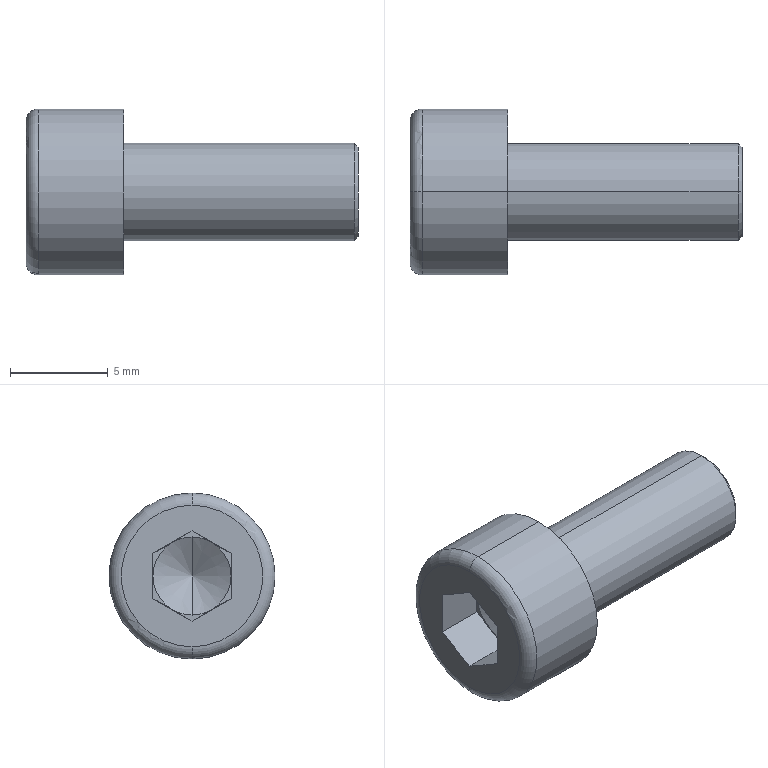Component | SolidWorks | hexagon socket head cap screws gb-3 | 1 solid | 25 faces | volume 477 mm3 | plane 15 | cone 4 | cylinder 4 | torus 2 | commonest cylinder face diameters 5 x2 8.5 x2